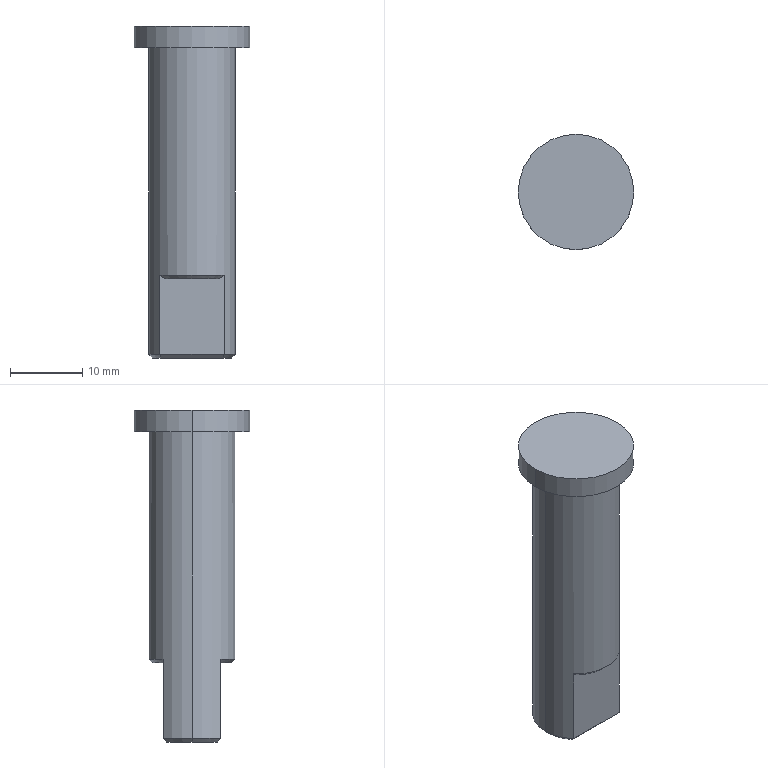Component | SolidWorks | TensioningWheel-2-1_XT-1-21-2-1 | 1 solid | 18 faces | box 16 x 16 x 46 mm | volume 5187 mm3 | plane 9 | cone 5 | cylinder 4 | commonest cylinder face diameters 16 x2 12 x2
STEP:
#1=CARTESIAN_POINT('',(20.966,-4.67,-5.945));
#2=VERTEX_POINT('',#1);
#3=CARTESIAN_POINT('',(21.015,-4.532,-5.945));
#4=VERTEX_POINT('',#3);
#5=CARTESIAN_POINT('',(21.183,-4.67,-5.945));
#6=DIRECTION('',(0.,0.,-1.));
#7=DIRECTION('',(-1.,0.,0.));
#8=AXIS2_PLACEMENT_3D('',#5,#6,#7);
#9=CIRCLE('',#8,0.2165);
#10=EDGE_CURVE('',#2,#4,#9,.T.);
#11=ORIENTED_EDGE('',*,*,#10,.F.);
#12=CARTESIAN_POINT('',(20.946,-4.67,-5.925));
#13=VERTEX_POINT('',#12);
#14=CARTESIAN_POINT('',(20.946,-4.67,-5.925));
#15=DIRECTION('',(-0.7071,0.,0.7071));
#16=VECTOR('',#15,39.37);
#17=LINE('',#14,#16);
#18=EDGE_CURVE('',#2,#13,#17,.T.);
#19=ORIENTED_EDGE('',*,*,#18,.T.);
#20=CARTESIAN_POINT('',(21.006,-4.512,-5.925));
#21=VERTEX_POINT('',#20);
#22=CARTESIAN_POINT('',(21.183,-4.67,-5.925));
#23=DIRECTION('',(0.,-0.,1.));
#24=DIRECTION('',(-1.,0.,0.));
#25=AXIS2_PLACEMENT_3D('',#22,#23,#24);
#26=CIRCLE('',#25,0.2362);
#27=EDGE_CURVE('',#21,#13,#26,.T.);
#28=ORIENTED_EDGE('',*,*,#27,.F.);
#29=CARTESIAN_POINT('',(21.006,-4.512,-5.925));
#30=CARTESIAN_POINT('',(21.009,-4.519,-5.932));
#31=CARTESIAN_POINT('',(21.012,-4.526,-5.938));
#32=CARTESIAN_POINT('',(21.015,-4.532,-5.945));
#33=B_SPLINE_CURVE_WITH_KNOTS('',3,(#29,#30,#31,#32),.UNSPECIFIED.,.F.,.F.,(4,4),(0.,0.0007434),.UNSPECIFIED.);
#34=EDGE_CURVE('',#21,#4,#33,.T.);
#35=ORIENTED_EDGE('',*,*,#34,.T.);
#36=EDGE_LOOP('',(#11,#19,#28,#35));
#37=FACE_OUTER_BOUND('',#36,.T.);
#38=CARTESIAN_POINT('',(21.183,-4.67,-5.925));
#39=DIRECTION('',(0.,-0.,1.));
#40=DIRECTION('',(-1.,0.,0.));
#41=AXIS2_PLACEMENT_3D('',#38,#39,#40);
#42=CONICAL_SURFACE('',#41,0.2362,0.7854);
#43=ADVANCED_FACE('',(#37),#42,.T.);
#44=CARTESIAN_POINT('',(20.868,-4.67,-4.252));
#45=VERTEX_POINT('',#44);
#46=CARTESIAN_POINT('',(21.497,-4.67,-4.252));
#47=VERTEX_POINT('',#46);
#48=CARTESIAN_POINT('',(21.183,-4.67,-4.252));
#49=DIRECTION('',(-0.,-0.,1.));
#50=DIRECTION('',(-1.,0.,0.));
#51=AXIS2_PLACEMENT_3D('',#48,#49,#50);
#52=CIRCLE('',#51,0.315);
#53=EDGE_CURVE('',#45,#47,#52,.T.);
#54=ORIENTED_EDGE('',*,*,#53,.T.);
#55=CARTESIAN_POINT('',(21.497,-4.67,-4.134));
#56=VERTEX_POINT('',#55);
#57=CARTESIAN_POINT('',(21.497,-4.67,-4.134));
#58=DIRECTION('',(-0.,-0.,1.));
#59=VECTOR('',#58,39.37);
#60=LINE('',#57,#59);
#61=EDGE_CURVE('',#47,#56,#60,.T.);
#62=ORIENTED_EDGE('',*,*,#61,.T.);
#63=CARTESIAN_POINT('',(20.868,-4.67,-4.134));
#64=VERTEX_POINT('',#63);
#65=CARTESIAN_POINT('',(21.183,-4.67,-4.134));
#66=DIRECTION('',(-0.,-0.,1.));
#67=DIRECTION('',(-1.,0.,0.));
#68=AXIS2_PLACEMENT_3D('',#65,#66,#67);
#69=CIRCLE('',#68,0.315);
#70=EDGE_CURVE('',#64,#56,#69,.T.);
#71=ORIENTED_EDGE('',*,*,#70,.F.);
#72=CARTESIAN_POINT('',(20.868,-4.67,-4.134));
#73=DIRECTION('',(-0.,-0.,1.));
#74=VECTOR('',#73,39.37);
#75=LINE('',#72,#74);
#76=EDGE_CURVE('',#45,#64,#75,.T.);
#77=ORIENTED_EDGE('',*,*,#76,.F.);
#78=EDGE_LOOP('',(#54,#62,#71,#77));
#79=FACE_OUTER_BOUND('',#78,.T.);
#80=CARTESIAN_POINT('',(21.183,-4.67,-4.134));
#81=DIRECTION('',(-0.,-0.,1.));
#82=DIRECTION('',(-1.,0.,0.));
#83=AXIS2_PLACEMENT_3D('',#80,#81,#82);
#84=CYLINDRICAL_SURFACE('',#83,0.315);
#85=ADVANCED_FACE('',(#79),#84,.T.);
#86=CARTESIAN_POINT('',(21.359,-4.827,-5.925));
#87=VERTEX_POINT('',#86);
#88=CARTESIAN_POINT('',(21.419,-4.67,-5.925));
#89=VERTEX_POINT('',#88);
#90=CARTESIAN_POINT('',(21.183,-4.67,-5.925));
#91=DIRECTION('',(0.,-0.,1.));
#92=DIRECTION('',(-1.,0.,0.));
#93=AXIS2_PLACEMENT_3D('',#90,#91,#92);
#94=CIRCLE('',#93,0.2362);
#95=EDGE_CURVE('',#87,#89,#94,.T.);
#96=ORIENTED_EDGE('',*,*,#95,.T.);
#97=CARTESIAN_POINT('',(21.419,-4.67,-4.252));
#98=VERTEX_POINT('',#97);
#99=CARTESIAN_POINT('',(21.419,-4.67,-4.134));
#100=DIRECTION('',(-0.,-0.,1.));
#101=VECTOR('',#100,39.37);
#102=LINE('',#99,#101);
#103=EDGE_CURVE('',#89,#98,#102,.T.);
#104=ORIENTED_EDGE('',*,*,#103,.T.);
#105=CARTESIAN_POINT('',(20.946,-4.67,-4.252));
#106=VERTEX_POINT('',#105);
#107=CARTESIAN_POINT('',(21.183,-4.67,-4.252));
#108=DIRECTION('',(-0.,-0.,1.));
#109=DIRECTION('',(-1.,0.,0.));
#110=AXIS2_PLACEMENT_3D('',#107,#108,#109);
#111=CIRCLE('',#110,0.2362);
#112=EDGE_CURVE('',#106,#98,#111,.T.);
#113=ORIENTED_EDGE('',*,*,#112,.F.);
#114=CARTESIAN_POINT('',(20.946,-4.67,-4.134));
#115=DIRECTION('',(-0.,-0.,1.));
#116=VECTOR('',#115,39.37);
#117=LINE('',#114,#116);
#118=EDGE_CURVE('',#13,#106,#117,.T.);
#119=ORIENTED_EDGE('',*,*,#118,.F.);
#120=CARTESIAN_POINT('',(21.006,-4.827,-5.925));
#121=VERTEX_POINT('',#120);
#122=CARTESIAN_POINT('',(21.183,-4.67,-5.925));
#123=DIRECTION('',(0.,-0.,1.));
#124=DIRECTION('',(-1.,0.,0.));
#125=AXIS2_PLACEMENT_3D('',#122,#123,#124);
#126=CIRCLE('',#125,0.2362);
#127=EDGE_CURVE('',#13,#121,#126,.T.);
#128=ORIENTED_EDGE('',*,*,#127,.T.);
#129=CARTESIAN_POINT('',(21.006,-4.827,-5.492));
#130=VERTEX_POINT('',#129);
#131=CARTESIAN_POINT('',(21.006,-4.827,-5.512));
#132=DIRECTION('',(0.,0.,-1.));
#133=VECTOR('',#132,39.37);
#134=LINE('',#131,#133);
#135=EDGE_CURVE('',#130,#121,#134,.T.);
#136=ORIENTED_EDGE('',*,*,#135,.F.);
#137=CARTESIAN_POINT('',(21.359,-4.827,-5.492));
#138=VERTEX_POINT('',#137);
#139=CARTESIAN_POINT('',(21.183,-4.67,-5.492));
#140=DIRECTION('',(-0.,-0.,1.));
#141=DIRECTION('',(1.,0.,0.));
#142=AXIS2_PLACEMENT_3D('',#139,#140,#141);
#143=CIRCLE('',#142,0.2362);
#144=EDGE_CURVE('',#130,#138,#143,.T.);
#145=ORIENTED_EDGE('',*,*,#144,.T.);
#146=CARTESIAN_POINT('',(21.359,-4.827,-5.512));
#147=DIRECTION('',(0.,0.,-1.));
#148=VECTOR('',#147,39.37);
#149=LINE('',#146,#148);
#150=EDGE_CURVE('',#138,#87,#149,.T.);
#151=ORIENTED_EDGE('',*,*,#150,.T.);
#152=EDGE_LOOP('',(#96,#104,#113,#119,#128,#136,#145,#151));
#153=FACE_OUTER_BOUND('',#152,.T.);
#154=CARTESIAN_POINT('',(21.183,-4.67,-4.134));
#155=DIRECTION('',(-0.,-0.,1.));
#156=DIRECTION('',(-1.,0.,0.));
#157=AXIS2_PLACEMENT_3D('',#154,#155,#156);
#158=CYLINDRICAL_SURFACE('',#157,0.2362);
#159=ADVANCED_FACE('',(#153),#158,.T.);
#160=ORIENTED_EDGE('',*,*,#70,.T.);
#161=CARTESIAN_POINT('',(21.183,-4.67,-4.134));
#162=DIRECTION('',(-0.,-0.,1.));
#163=DIRECTION('',(-1.,0.,0.));
#164=AXIS2_PLACEMENT_3D('',#161,#162,#163);
#165=CIRCLE('',#164,0.315);
#166=EDGE_CURVE('',#56,#64,#165,.T.);
#167=ORIENTED_EDGE('',*,*,#166,.T.);
#168=EDGE_LOOP('',(#160,#167));
#169=FACE_OUTER_BOUND('',#168,.T.);
#170=CARTESIAN_POINT('',(21.497,-4.67,-4.134));
#171=DIRECTION('',(0.,0.,-1.));
#172=DIRECTION('',(1.,-0.,0.));
#173=AXIS2_PLACEMENT_3D('',#170,#171,#172);
#174=PLANE('',#173);
#175=ADVANCED_FACE('',(#169),#174,.F.);
#176=CARTESIAN_POINT('',(21.35,-4.808,-5.945));
#177=VERTEX_POINT('',#176);
#178=CARTESIAN_POINT('',(21.015,-4.808,-5.945));
#179=VERTEX_POINT('',#178);
#180=CARTESIAN_POINT('',(21.183,-4.808,-5.945));
#181=DIRECTION('',(-1.,0.,-0.));
#182=VECTOR('',#181,39.37);
#183=LINE('',#180,#182);
#184=EDGE_CURVE('',#177,#179,#183,.T.);
#185=ORIENTED_EDGE('',*,*,#184,.T.);
#186=CARTESIAN_POINT('',(21.183,-4.67,-5.945));
#187=DIRECTION('',(0.,0.,-1.));
#188=DIRECTION('',(-1.,-0.,0.));
#189=AXIS2_PLACEMENT_3D('',#186,#187,#188);
#190=CIRCLE('',#189,0.2165);
#191=EDGE_CURVE('',#179,#2,#190,.T.);
#192=ORIENTED_EDGE('',*,*,#191,.T.);
#193=ORIENTED_EDGE('',*,*,#10,.T.);
#194=CARTESIAN_POINT('',(21.35,-4.532,-5.945));
#195=VERTEX_POINT('',#194);
#196=CARTESIAN_POINT('',(21.183,-4.532,-5.945));
#197=DIRECTION('',(1.,-0.,0.));
#198=VECTOR('',#197,39.37);
#199=LINE('',#196,#198);
#200=EDGE_CURVE('',#4,#195,#199,.T.);
#201=ORIENTED_EDGE('',*,*,#200,.T.);
#202=CARTESIAN_POINT('',(21.183,-4.67,-5.945));
#203=DIRECTION('',(0.,0.,-1.));
#204=DIRECTION('',(-1.,0.,0.));
#205=AXIS2_PLACEMENT_3D('',#202,#203,#204);
#206=CIRCLE('',#205,0.2165);
#207=EDGE_CURVE('',#195,#177,#206,.T.);
#208=ORIENTED_EDGE('',*,*,#207,.T.);
#209=EDGE_LOOP('',(#185,#192,#193,#201,#208));
#210=FACE_OUTER_BOUND('',#209,.T.);
#211=CARTESIAN_POINT('',(21.183,-4.67,-5.945));
#212=DIRECTION('',(-0.,-0.,1.));
#213=DIRECTION('',(-1.,0.,-0.));
#214=AXIS2_PLACEMENT_3D('',#211,#212,#213);
#215=PLANE('',#214);
#216=ADVANCED_FACE('',(#210),#215,.F.);
#217=ORIENTED_EDGE('',*,*,#103,.F.);
#218=CARTESIAN_POINT('',(21.359,-4.512,-5.925));
#219=VERTEX_POINT('',#218);
#220=CARTESIAN_POINT('',(21.183,-4.67,-5.925));
#221=DIRECTION('',(0.,-0.,1.));
#222=DIRECTION('',(-1.,0.,0.));
#223=AXIS2_PLACEMENT_3D('',#220,#221,#222);
#224=CIRCLE('',#223,0.2362);
#225=EDGE_CURVE('',#89,#219,#224,.T.);
#226=ORIENTED_EDGE('',*,*,#225,.T.);
#227=CARTESIAN_POINT('',(21.359,-4.512,-5.492));
#228=VERTEX_POINT('',#227);
#229=CARTESIAN_POINT('',(21.359,-4.512,-5.512));
#230=DIRECTION('',(0.,0.,-1.));
#231=VECTOR('',#230,39.37);
#232=LINE('',#229,#231);
#233=EDGE_CURVE('',#228,#219,#232,.T.);
#234=ORIENTED_EDGE('',*,*,#233,.F.);
#235=CARTESIAN_POINT('',(21.006,-4.512,-5.492));
#236=VERTEX_POINT('',#235);
#237=CARTESIAN_POINT('',(21.183,-4.67,-5.492));
#238=DIRECTION('',(-0.,-0.,1.));
#239=DIRECTION('',(1.,0.,0.));
#240=AXIS2_PLACEMENT_3D('',#237,#238,#239);
#241=CIRCLE('',#240,0.2362);
#242=EDGE_CURVE('',#228,#236,#241,.T.);
#243=ORIENTED_EDGE('',*,*,#242,.T.);
#244=CARTESIAN_POINT('',(21.006,-4.512,-5.512));
#245=DIRECTION('',(0.,0.,-1.));
#246=VECTOR('',#245,39.37);
#247=LINE('',#244,#246);
#248=EDGE_CURVE('',#236,#21,#247,.T.);
#249=ORIENTED_EDGE('',*,*,#248,.T.);
#250=ORIENTED_EDGE('',*,*,#27,.T.);
#251=ORIENTED_EDGE('',*,*,#118,.T.);
#252=CARTESIAN_POINT('',(21.183,-4.67,-4.252));
#253=DIRECTION('',(-0.,-0.,1.));
#254=DIRECTION('',(-1.,0.,0.));
#255=AXIS2_PLACEMENT_3D('',#252,#253,#254);
#256=CIRCLE('',#255,0.2362);
#257=EDGE_CURVE('',#98,#106,#256,.T.);
#258=ORIENTED_EDGE('',*,*,#257,.F.);
#259=EDGE_LOOP('',(#217,#226,#234,#243,#249,#250,#251,#258));
#260=FACE_OUTER_BOUND('',#259,.T.);
#261=CARTESIAN_POINT('',(21.183,-4.67,-4.134));
#262=DIRECTION('',(-0.,-0.,1.));
#263=DIRECTION('',(-1.,0.,0.));
#264=AXIS2_PLACEMENT_3D('',#261,#262,#263);
#265=CYLINDRICAL_SURFACE('',#264,0.2362);
#266=ADVANCED_FACE('',(#260),#265,.T.);
#267=ORIENTED_EDGE('',*,*,#53,.F.);
#268=CARTESIAN_POINT('',(21.183,-4.67,-4.252));
#269=DIRECTION('',(-0.,-0.,1.));
#270=DIRECTION('',(-1.,0.,0.));
#271=AXIS2_PLACEMENT_3D('',#268,#269,#270);
#272=CIRCLE('',#271,0.315);
#273=EDGE_CURVE('',#47,#45,#272,.T.);
#274=ORIENTED_EDGE('',*,*,#273,.F.);
#275=EDGE_LOOP('',(#267,#274));
#276=FACE_OUTER_BOUND('',#275,.T.);
#277=ORIENTED_EDGE('',*,*,#112,.T.);
#278=ORIENTED_EDGE('',*,*,#257,.T.);
#279=EDGE_LOOP('',(#277,#278));
#280=FACE_BOUND('',#279,.T.);
#281=CARTESIAN_POINT('',(21.419,-4.67,-4.252));
#282=DIRECTION('',(-0.,-0.,1.));
#283=DIRECTION('',(-1.,0.,-0.));
#284=AXIS2_PLACEMENT_3D('',#281,#282,#283);
#285=PLANE('',#284);
#286=ADVANCED_FACE('',(#276,#280),#285,.F.);
#287=ORIENTED_EDGE('',*,*,#61,.F.);
#288=ORIENTED_EDGE('',*,*,#273,.T.);
#289=ORIENTED_EDGE('',*,*,#76,.T.);
#290=ORIENTED_EDGE('',*,*,#166,.F.);
#291=EDGE_LOOP('',(#287,#288,#289,#290));
#292=FACE_OUTER_BOUND('',#291,.T.);
#293=CARTESIAN_POINT('',(21.183,-4.67,-4.134));
#294=DIRECTION('',(-0.,-0.,1.));
#295=DIRECTION('',(-1.,0.,0.));
#296=AXIS2_PLACEMENT_3D('',#293,#294,#295);
#297=CYLINDRICAL_SURFACE('',#296,0.315);
#298=ADVANCED_FACE('',(#292),#297,.T.);
#299=ORIENTED_EDGE('',*,*,#135,.T.);
#300=CARTESIAN_POINT('',(21.006,-4.827,-5.925));
#301=DIRECTION('',(1.,-0.,0.));
#302=VECTOR('',#301,39.37);
#303=LINE('',#300,#302);
#304=EDGE_CURVE('',#121,#87,#303,.T.);
#305=ORIENTED_EDGE('',*,*,#304,.T.);
#306=ORIENTED_EDGE('',*,*,#150,.F.);
#307=CARTESIAN_POINT('',(21.331,-4.827,-5.512));
#308=VERTEX_POINT('',#307);
#309=CARTESIAN_POINT('',(21.359,-4.827,-5.492));
#310=CARTESIAN_POINT('',(21.35,-4.827,-5.499));
#311=CARTESIAN_POINT('',(21.34,-4.827,-5.505));
#312=CARTESIAN_POINT('',(21.331,-4.827,-5.512));
#313=B_SPLINE_CURVE_WITH_KNOTS('',3,(#309,#310,#311,#312),.UNSPECIFIED.,.F.,.F.,(4,4),(0.,0.000858),.UNSPECIFIED.);
#314=EDGE_CURVE('',#138,#308,#313,.T.);
#315=ORIENTED_EDGE('',*,*,#314,.T.);
#316=CARTESIAN_POINT('',(21.034,-4.827,-5.512));
#317=VERTEX_POINT('',#316);
#318=CARTESIAN_POINT('',(21.006,-4.827,-5.512));
#319=DIRECTION('',(1.,-0.,-0.));
#320=VECTOR('',#319,39.37);
#321=LINE('',#318,#320);
#322=EDGE_CURVE('',#317,#308,#321,.T.);
#323=ORIENTED_EDGE('',*,*,#322,.F.);
#324=CARTESIAN_POINT('',(21.034,-4.827,-5.512));
#325=CARTESIAN_POINT('',(21.025,-4.827,-5.505));
#326=CARTESIAN_POINT('',(21.015,-4.827,-5.499));
#327=CARTESIAN_POINT('',(21.006,-4.827,-5.492));
#328=B_SPLINE_CURVE_WITH_KNOTS('',3,(#324,#325,#326,#327),.UNSPECIFIED.,.F.,.F.,(4,4),(0.,0.000858),.UNSPECIFIED.);
#329=EDGE_CURVE('',#317,#130,#328,.T.);
#330=ORIENTED_EDGE('',*,*,#329,.T.);
#331=EDGE_LOOP('',(#299,#305,#306,#315,#323,#330));
#332=FACE_OUTER_BOUND('',#331,.T.);
#333=CARTESIAN_POINT('',(21.006,-4.827,-5.512));
#334=DIRECTION('',(0.,1.,0.));
#335=DIRECTION('',(-1.,0.,0.));
#336=AXIS2_PLACEMENT_3D('',#333,#334,#335);
#337=PLANE('',#336);
#338=ADVANCED_FACE('',(#332),#337,.F.);
#339=ORIENTED_EDGE('',*,*,#322,.T.);
#340=CARTESIAN_POINT('',(21.183,-4.67,-5.512));
#341=DIRECTION('',(0.,0.,-1.));
#342=DIRECTION('',(1.,0.,0.));
#343=AXIS2_PLACEMENT_3D('',#340,#341,#342);
#344=CIRCLE('',#343,0.2165);
#345=EDGE_CURVE('',#308,#317,#344,.T.);
#346=ORIENTED_EDGE('',*,*,#345,.T.);
#347=EDGE_LOOP('',(#339,#346));
#348=FACE_OUTER_BOUND('',#347,.T.);
#349=CARTESIAN_POINT('',(21.183,-4.67,-5.512));
#350=DIRECTION('',(0.,0.,-1.));
#351=DIRECTION('',(1.,-0.,0.));
#352=AXIS2_PLACEMENT_3D('',#349,#350,#351);
#353=PLANE('',#352);
#354=ADVANCED_FACE('',(#348),#353,.T.);
#355=ORIENTED_EDGE('',*,*,#233,.T.);
#356=CARTESIAN_POINT('',(21.006,-4.512,-5.925));
#357=DIRECTION('',(-1.,0.,-0.));
#358=VECTOR('',#357,39.37);
#359=LINE('',#356,#358);
#360=EDGE_CURVE('',#219,#21,#359,.T.);
#361=ORIENTED_EDGE('',*,*,#360,.T.);
#362=ORIENTED_EDGE('',*,*,#248,.F.);
#363=CARTESIAN_POINT('',(21.034,-4.512,-5.512));
#364=VERTEX_POINT('',#363);
#365=CARTESIAN_POINT('',(21.006,-4.512,-5.492));
#366=CARTESIAN_POINT('',(21.015,-4.512,-5.499));
#367=CARTESIAN_POINT('',(21.025,-4.512,-5.505));
#368=CARTESIAN_POINT('',(21.034,-4.512,-5.512));
#369=B_SPLINE_CURVE_WITH_KNOTS('',3,(#365,#366,#367,#368),.UNSPECIFIED.,.F.,.F.,(4,4),(0.,0.000858),.UNSPECIFIED.);
#370=EDGE_CURVE('',#236,#364,#369,.T.);
#371=ORIENTED_EDGE('',*,*,#370,.T.);
#372=CARTESIAN_POINT('',(21.331,-4.512,-5.512));
#373=VERTEX_POINT('',#372);
#374=CARTESIAN_POINT('',(21.006,-4.512,-5.512));
#375=DIRECTION('',(-1.,0.,0.));
#376=VECTOR('',#375,39.37);
#377=LINE('',#374,#376);
#378=EDGE_CURVE('',#373,#364,#377,.T.);
#379=ORIENTED_EDGE('',*,*,#378,.F.);
#380=CARTESIAN_POINT('',(21.331,-4.512,-5.512));
#381=CARTESIAN_POINT('',(21.34,-4.512,-5.505));
#382=CARTESIAN_POINT('',(21.35,-4.512,-5.499));
#383=CARTESIAN_POINT('',(21.359,-4.512,-5.492));
#384=B_SPLINE_CURVE_WITH_KNOTS('',3,(#380,#381,#382,#383),.UNSPECIFIED.,.F.,.F.,(4,4),(0.,0.000858),.UNSPECIFIED.);
#385=EDGE_CURVE('',#373,#228,#384,.T.);
#386=ORIENTED_EDGE('',*,*,#385,.T.);
#387=EDGE_LOOP('',(#355,#361,#362,#371,#379,#386));
#388=FACE_OUTER_BOUND('',#387,.T.);
#389=CARTESIAN_POINT('',(21.006,-4.512,-5.512));
#390=DIRECTION('',(-0.,-1.,-0.));
#391=DIRECTION('',(1.,-0.,-0.));
#392=AXIS2_PLACEMENT_3D('',#389,#390,#391);
#393=PLANE('',#392);
#394=ADVANCED_FACE('',(#388),#393,.F.);
#395=ORIENTED_EDGE('',*,*,#378,.T.);
#396=CARTESIAN_POINT('',(21.183,-4.67,-5.512));
#397=DIRECTION('',(0.,0.,-1.));
#398=DIRECTION('',(1.,0.,0.));
#399=AXIS2_PLACEMENT_3D('',#396,#397,#398);
#400=CIRCLE('',#399,0.2165);
#401=EDGE_CURVE('',#364,#373,#400,.T.);
#402=ORIENTED_EDGE('',*,*,#401,.T.);
#403=EDGE_LOOP('',(#395,#402));
#404=FACE_OUTER_BOUND('',#403,.T.);
#405=CARTESIAN_POINT('',(21.183,-4.67,-5.512));
#406=DIRECTION('',(0.,0.,-1.));
#407=DIRECTION('',(1.,-0.,0.));
#408=AXIS2_PLACEMENT_3D('',#405,#406,#407);
#409=PLANE('',#408);
#410=ADVANCED_FACE('',(#404),#409,.T.);
#411=CARTESIAN_POINT('',(21.35,-4.808,-5.945));
#412=CARTESIAN_POINT('',(21.353,-4.814,-5.938));
#413=CARTESIAN_POINT('',(21.356,-4.821,-5.932));
#414=CARTESIAN_POINT('',(21.359,-4.827,-5.925));
#415=B_SPLINE_CURVE_WITH_KNOTS('',3,(#411,#412,#413,#414),.UNSPECIFIED.,.F.,.F.,(4,4),(0.,0.0007434),.UNSPECIFIED.);
#416=EDGE_CURVE('',#177,#87,#415,.T.);
#417=ORIENTED_EDGE('',*,*,#416,.F.);
#418=ORIENTED_EDGE('',*,*,#207,.F.);
#419=CARTESIAN_POINT('',(21.359,-4.512,-5.925));
#420=CARTESIAN_POINT('',(21.356,-4.519,-5.932));
#421=CARTESIAN_POINT('',(21.353,-4.526,-5.938));
#422=CARTESIAN_POINT('',(21.35,-4.532,-5.945));
#423=B_SPLINE_CURVE_WITH_KNOTS('',3,(#419,#420,#421,#422),.UNSPECIFIED.,.F.,.F.,(4,4),(0.,0.0007434),.UNSPECIFIED.);
#424=EDGE_CURVE('',#219,#195,#423,.T.);
#425=ORIENTED_EDGE('',*,*,#424,.F.);
#426=ORIENTED_EDGE('',*,*,#225,.F.);
#427=ORIENTED_EDGE('',*,*,#95,.F.);
#428=EDGE_LOOP('',(#417,#418,#425,#426,#427));
#429=FACE_OUTER_BOUND('',#428,.T.);
#430=CARTESIAN_POINT('',(21.183,-4.67,-5.925));
#431=DIRECTION('',(0.,-0.,1.));
#432=DIRECTION('',(-1.,0.,0.));
#433=AXIS2_PLACEMENT_3D('',#430,#431,#432);
#434=CONICAL_SURFACE('',#433,0.2362,0.7854);
#435=ADVANCED_FACE('',(#429),#434,.T.);
#436=ORIENTED_EDGE('',*,*,#424,.T.);
#437=ORIENTED_EDGE('',*,*,#200,.F.);
#438=ORIENTED_EDGE('',*,*,#34,.F.);
#439=ORIENTED_EDGE('',*,*,#360,.F.);
#440=EDGE_LOOP('',(#436,#437,#438,#439));
#441=FACE_OUTER_BOUND('',#440,.T.);
#442=CARTESIAN_POINT('',(21.006,-4.512,-5.925));
#443=DIRECTION('',(-0.,-0.7071,0.7071));
#444=DIRECTION('',(-1.,0.,-0.));
#445=AXIS2_PLACEMENT_3D('',#442,#443,#444);
#446=PLANE('',#445);
#447=ADVANCED_FACE('',(#441),#446,.F.);
#448=ORIENTED_EDGE('',*,*,#416,.T.);
#449=ORIENTED_EDGE('',*,*,#304,.F.);
#450=CARTESIAN_POINT('',(21.015,-4.808,-5.945));
#451=CARTESIAN_POINT('',(21.012,-4.814,-5.938));
#452=CARTESIAN_POINT('',(21.009,-4.821,-5.932));
#453=CARTESIAN_POINT('',(21.006,-4.827,-5.925));
#454=B_SPLINE_CURVE_WITH_KNOTS('',3,(#450,#451,#452,#453),.UNSPECIFIED.,.F.,.F.,(4,4),(0.,0.0007434),.UNSPECIFIED.);
#455=EDGE_CURVE('',#179,#121,#454,.T.);
#456=ORIENTED_EDGE('',*,*,#455,.F.);
#457=ORIENTED_EDGE('',*,*,#184,.F.);
#458=EDGE_LOOP('',(#448,#449,#456,#457));
#459=FACE_OUTER_BOUND('',#458,.T.);
#460=CARTESIAN_POINT('',(21.006,-4.827,-5.925));
#461=DIRECTION('',(0.,0.7071,0.7071));
#462=DIRECTION('',(1.,-0.,0.));
#463=AXIS2_PLACEMENT_3D('',#460,#461,#462);
#464=PLANE('',#463);
#465=ADVANCED_FACE('',(#459),#464,.F.);
#466=ORIENTED_EDGE('',*,*,#18,.F.);
#467=ORIENTED_EDGE('',*,*,#191,.F.);
#468=ORIENTED_EDGE('',*,*,#455,.T.);
#469=ORIENTED_EDGE('',*,*,#127,.F.);
#470=EDGE_LOOP('',(#466,#467,#468,#469));
#471=FACE_OUTER_BOUND('',#470,.T.);
#472=CARTESIAN_POINT('',(21.183,-4.67,-5.925));
#473=DIRECTION('',(0.,-0.,1.));
#474=DIRECTION('',(-1.,0.,0.));
#475=AXIS2_PLACEMENT_3D('',#472,#473,#474);
#476=CONICAL_SURFACE('',#475,0.2362,0.7854);
#477=ADVANCED_FACE('',(#471),#476,.T.);
#478=ORIENTED_EDGE('',*,*,#370,.F.);
#479=ORIENTED_EDGE('',*,*,#242,.F.);
#480=ORIENTED_EDGE('',*,*,#385,.F.);
#481=ORIENTED_EDGE('',*,*,#401,.F.);
#482=EDGE_LOOP('',(#478,#479,#480,#481));
#483=FACE_OUTER_BOUND('',#482,.T.);
#484=CARTESIAN_POINT('',(21.183,-4.67,-5.512));
#485=DIRECTION('',(-0.,-0.,1.));
#486=DIRECTION('',(-1.,0.,0.));
#487=AXIS2_PLACEMENT_3D('',#484,#485,#486);
#488=CONICAL_SURFACE('',#487,0.2165,0.7854);
#489=ADVANCED_FACE('',(#483),#488,.T.);
#490=ORIENTED_EDGE('',*,*,#314,.F.);
#491=ORIENTED_EDGE('',*,*,#144,.F.);
#492=ORIENTED_EDGE('',*,*,#329,.F.);
#493=ORIENTED_EDGE('',*,*,#345,.F.);
#494=EDGE_LOOP('',(#490,#491,#492,#493));
#495=FACE_OUTER_BOUND('',#494,.T.);
#496=CARTESIAN_POINT('',(21.183,-4.67,-5.512));
#497=DIRECTION('',(-0.,-0.,1.));
#498=DIRECTION('',(-1.,0.,0.));
#499=AXIS2_PLACEMENT_3D('',#496,#497,#498);
#500=CONICAL_SURFACE('',#499,0.2165,0.7854);
#501=ADVANCED_FACE('',(#495),#500,.T.);
#502=CLOSED_SHELL('',(#43,#85,#159,#175,#216,#266,#286,#298,#338,#354,#394,#410,#435,#447,#465,#477,#489,#501));
#503=MANIFOLD_SOLID_BREP('',#502);
#504=CARTESIAN_POINT('',(0.,0.,0.));
#505=DIRECTION('',(0.,0.,1.));
#506=DIRECTION('',(1.,0.,0.));
#507=AXIS2_PLACEMENT_3D('',#504,#505,#506);
#508=(LENGTH_UNIT()NAMED_UNIT(*)SI_UNIT($,.METRE.));
#509=LENGTH_MEASURE_WITH_UNIT(LENGTH_MEASURE(0.0254),#508);
#510=DIMENSIONAL_EXPONENTS(1.,0.,0.,0.,0.,0.,0.);
#511=(CONVERSION_BASED_UNIT('',#509)LENGTH_UNIT()NAMED_UNIT(#510));
#512=UNCERTAINTY_MEASURE_WITH_UNIT(LENGTH_MEASURE(0.00001),#511,'','');
#513=(NAMED_UNIT(*)PLANE_ANGLE_UNIT()SI_UNIT($,.RADIAN.));
#514=(NAMED_UNIT(*)SI_UNIT($,.STERADIAN.)SOLID_ANGLE_UNIT());
#515=(GEOMETRIC_REPRESENTATION_CONTEXT(3)GLOBAL_UNCERTAINTY_ASSIGNED_CONTEXT((#512))GLOBAL_UNIT_ASSIGNED_CONTEXT((#511,#513,#514))REPRESENTATION_CONTEXT('',''));
#516=ADVANCED_BREP_SHAPE_REPRESENTATION('',(#503,#507),#515);
#517=COLOUR_RGB('',0.7922,0.8196,0.9333);
#518=FILL_AREA_STYLE_COLOUR('',#517);
#519=FILL_AREA_STYLE('',(#518));
#520=SURFACE_STYLE_FILL_AREA(#519);
#521=SURFACE_SIDE_STYLE('',(#520));
#522=SURFACE_STYLE_USAGE(.BOTH.,#521);
#523=PRESENTATION_STYLE_ASSIGNMENT((#522));
#524=STYLED_ITEM('',(#523),#503);
#525=PRESENTATION_LAYER_ASSIGNMENT('','',(#524));
#526=(LENGTH_UNIT()NAMED_UNIT(*)SI_UNIT($,.METRE.));
#527=LENGTH_MEASURE_WITH_UNIT(LENGTH_MEASURE(0.0254),#526);
#528=DIMENSIONAL_EXPONENTS(1.,0.,0.,0.,0.,0.,0.);
#529=(CONVERSION_BASED_UNIT('',#527)LENGTH_UNIT()NAMED_UNIT(#528));
#530=UNCERTAINTY_MEASURE_WITH_UNIT(LENGTH_MEASURE(0.00001),#529,'','');
#531=(NAMED_UNIT(*)PLANE_ANGLE_UNIT()SI_UNIT($,.RADIAN.));
#532=(NAMED_UNIT(*)SI_UNIT($,.STERADIAN.)SOLID_ANGLE_UNIT());
#533=(GEOMETRIC_REPRESENTATION_CONTEXT(3)GLOBAL_UNCERTAINTY_ASSIGNED_CONTEXT((#530))GLOBAL_UNIT_ASSIGNED_CONTEXT((#529,#531,#532))REPRESENTATION_CONTEXT('',''));
#534=MECHANICAL_DESIGN_GEOMETRIC_PRESENTATION_REPRESENTATION('',(#524),#533);